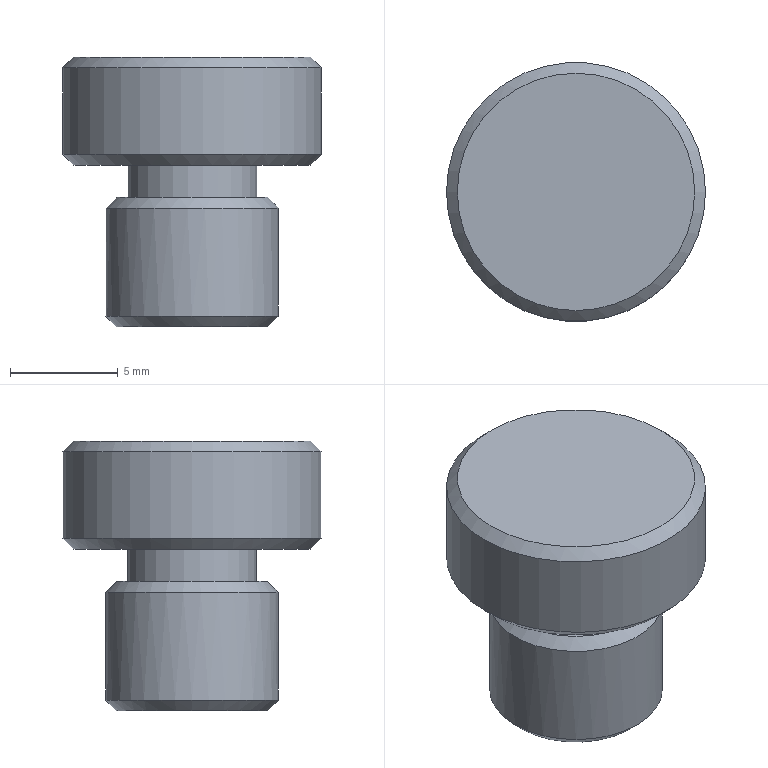Component | NX | SUPPORT_PIN_4 | 1 solid | 11 faces | box 12 x 12 x 12.5 mm | volume 894 mm3 | plane 4 | cone 4 | cylinder 3 | commonest cylinder face diameters 8 x1 6 x1 12 x1
STEP:
#1=CARTESIAN_POINT('',(0.,0.,0.));
#2=DIRECTION('',(0.,0.,1.));
#3=DIRECTION('',(1.,0.,0.));
#4=AXIS2_PLACEMENT_3D('',#1,#2,#3);
#5=CARTESIAN_POINT('',(405.601,61.,87.5));
#6=VERTEX_POINT('',#5);
#7=CARTESIAN_POINT('',(402.101,61.,87.5));
#8=DIRECTION('',(0.,0.,1.));
#9=DIRECTION('',(1.,0.,0.));
#10=AXIS2_PLACEMENT_3D('',#7,#8,#9);
#11=CIRCLE('',#10,3.5);
#12=CARTESIAN_POINT('',(402.101,61.,87.5));
#13=DIRECTION('',(0.,0.,1.));
#14=DIRECTION('',(1.,0.,0.));
#15=AXIS2_PLACEMENT_3D('',#12,#13,#14);
#16=PLANE('',#15);
#17=CARTESIAN_POINT('',(0.,0.));
#18=DIRECTION('',(1.,0.));
#19=AXIS2_PLACEMENT_2D('',#17,#18);
#20=CIRCLE('',#19,3.5);
#21=(GEOMETRIC_REPRESENTATION_CONTEXT(2)PARAMETRIC_REPRESENTATION_CONTEXT()REPRESENTATION_CONTEXT('',''));
#22=DEFINITIONAL_REPRESENTATION('',(#20),#21);
#23=PCURVE('',#16,#22);
#24=CARTESIAN_POINT('',(402.101,61.,87.));
#25=DIRECTION('',(0.,0.,-1.));
#26=DIRECTION('',(-1.,0.,0.));
#27=AXIS2_PLACEMENT_3D('',#24,#25,#26);
#28=CONICAL_SURFACE('',#27,4.,0.7854);
#29=CARTESIAN_POINT('',(9.425,-0.5));
#30=DIRECTION('',(-1.,0.));
#31=VECTOR('',#30,1.);
#32=LINE('',#29,#31);
#33=(GEOMETRIC_REPRESENTATION_CONTEXT(2)PARAMETRIC_REPRESENTATION_CONTEXT()REPRESENTATION_CONTEXT('',''));
#34=DEFINITIONAL_REPRESENTATION('',(#32),#33);
#35=PCURVE('',#28,#34);
#36=SURFACE_CURVE('',#11,(#23,#35),.PCURVE_S1.);
#37=EDGE_CURVE('',#6,#6,#36,.T.);
#38=ORIENTED_EDGE('',*,*,#37,.T.);
#39=EDGE_LOOP('',(#38));
#40=FACE_BOUND('',#39,.T.);
#41=CARTESIAN_POINT('',(405.101,61.,87.5));
#42=VERTEX_POINT('',#41);
#43=CARTESIAN_POINT('',(402.101,61.,87.5));
#44=DIRECTION('',(0.,0.,1.));
#45=DIRECTION('',(1.,0.,0.));
#46=AXIS2_PLACEMENT_3D('',#43,#44,#45);
#47=CIRCLE('',#46,3.);
#48=CARTESIAN_POINT('',(0.,0.));
#49=DIRECTION('',(1.,0.));
#50=AXIS2_PLACEMENT_2D('',#48,#49);
#51=CIRCLE('',#50,3.);
#52=(GEOMETRIC_REPRESENTATION_CONTEXT(2)PARAMETRIC_REPRESENTATION_CONTEXT()REPRESENTATION_CONTEXT('',''));
#53=DEFINITIONAL_REPRESENTATION('',(#51),#52);
#54=PCURVE('',#16,#53);
#55=CARTESIAN_POINT('',(402.101,61.,87.5));
#56=DIRECTION('',(0.,0.,1.));
#57=DIRECTION('',(1.,0.,0.));
#58=AXIS2_PLACEMENT_3D('',#55,#56,#57);
#59=CYLINDRICAL_SURFACE('',#58,3.);
#60=CARTESIAN_POINT('',(0.,0.));
#61=DIRECTION('',(1.,0.));
#62=VECTOR('',#61,1.);
#63=LINE('',#60,#62);
#64=(GEOMETRIC_REPRESENTATION_CONTEXT(2)PARAMETRIC_REPRESENTATION_CONTEXT()REPRESENTATION_CONTEXT('',''));
#65=DEFINITIONAL_REPRESENTATION('',(#63),#64);
#66=PCURVE('',#59,#65);
#67=SURFACE_CURVE('',#47,(#54,#66),.PCURVE_S1.);
#68=EDGE_CURVE('',#42,#42,#67,.T.);
#69=ORIENTED_EDGE('',*,*,#68,.F.);
#70=EDGE_LOOP('',(#69));
#71=FACE_BOUND('',#70,.T.);
#72=ADVANCED_FACE('',(#40,#71),#16,.T.);
#73=CARTESIAN_POINT('',(398.601,61.,81.5));
#74=VERTEX_POINT('',#73);
#75=CARTESIAN_POINT('',(402.101,61.,81.5));
#76=DIRECTION('',(0.,0.,-1.));
#77=DIRECTION('',(-1.,0.,0.));
#78=AXIS2_PLACEMENT_3D('',#75,#76,#77);
#79=CIRCLE('',#78,3.5);
#80=CARTESIAN_POINT('',(402.101,61.,81.5));
#81=DIRECTION('',(0.,0.,-1.));
#82=DIRECTION('',(-1.,0.,0.));
#83=AXIS2_PLACEMENT_3D('',#80,#81,#82);
#84=PLANE('',#83);
#85=CARTESIAN_POINT('',(0.,0.));
#86=DIRECTION('',(1.,0.));
#87=AXIS2_PLACEMENT_2D('',#85,#86);
#88=CIRCLE('',#87,3.5);
#89=(GEOMETRIC_REPRESENTATION_CONTEXT(2)PARAMETRIC_REPRESENTATION_CONTEXT()REPRESENTATION_CONTEXT('',''));
#90=DEFINITIONAL_REPRESENTATION('',(#88),#89);
#91=PCURVE('',#84,#90);
#92=CARTESIAN_POINT('',(402.101,61.,82.));
#93=DIRECTION('',(0.,0.,1.));
#94=DIRECTION('',(1.,0.,0.));
#95=AXIS2_PLACEMENT_3D('',#92,#93,#94);
#96=CONICAL_SURFACE('',#95,4.,0.7854);
#97=CARTESIAN_POINT('',(9.425,-0.5));
#98=DIRECTION('',(-1.,0.));
#99=VECTOR('',#98,1.);
#100=LINE('',#97,#99);
#101=(GEOMETRIC_REPRESENTATION_CONTEXT(2)PARAMETRIC_REPRESENTATION_CONTEXT()REPRESENTATION_CONTEXT('',''));
#102=DEFINITIONAL_REPRESENTATION('',(#100),#101);
#103=PCURVE('',#96,#102);
#104=SURFACE_CURVE('',#79,(#91,#103),.PCURVE_S1.);
#105=EDGE_CURVE('',#74,#74,#104,.T.);
#106=ORIENTED_EDGE('',*,*,#105,.T.);
#107=EDGE_LOOP('',(#106));
#108=FACE_BOUND('',#107,.T.);
#109=ADVANCED_FACE('',(#108),#84,.T.);
#110=CARTESIAN_POINT('',(398.101,61.,82.));
#111=VERTEX_POINT('',#110);
#112=CARTESIAN_POINT('',(406.101,61.,82.));
#113=VERTEX_POINT('',#112);
#114=CARTESIAN_POINT('',(402.101,61.,82.));
#115=DIRECTION('',(0.,0.,1.));
#116=DIRECTION('',(-1.,0.,0.));
#117=AXIS2_PLACEMENT_3D('',#114,#115,#116);
#118=CIRCLE('',#117,4.);
#119=CARTESIAN_POINT('',(402.101,61.,81.5));
#120=DIRECTION('',(0.,0.,1.));
#121=DIRECTION('',(1.,0.,0.));
#122=AXIS2_PLACEMENT_3D('',#119,#120,#121);
#123=CYLINDRICAL_SURFACE('',#122,4.);
#124=CARTESIAN_POINT('',(3.142,0.5));
#125=DIRECTION('',(1.,0.));
#126=VECTOR('',#125,1.);
#127=LINE('',#124,#126);
#128=(GEOMETRIC_REPRESENTATION_CONTEXT(2)PARAMETRIC_REPRESENTATION_CONTEXT()REPRESENTATION_CONTEXT('',''));
#129=DEFINITIONAL_REPRESENTATION('',(#127),#128);
#130=PCURVE('',#123,#129);
#131=CARTESIAN_POINT('',(3.142,0.));
#132=DIRECTION('',(1.,0.));
#133=VECTOR('',#132,1.);
#134=LINE('',#131,#133);
#135=(GEOMETRIC_REPRESENTATION_CONTEXT(2)PARAMETRIC_REPRESENTATION_CONTEXT()REPRESENTATION_CONTEXT('',''));
#136=DEFINITIONAL_REPRESENTATION('',(#134),#135);
#137=PCURVE('',#96,#136);
#138=SURFACE_CURVE('',#118,(#130,#137),.PCURVE_S1.);
#139=EDGE_CURVE('',#111,#113,#138,.T.);
#140=ORIENTED_EDGE('',*,*,#139,.T.);
#141=CARTESIAN_POINT('',(406.101,61.,87.));
#142=VERTEX_POINT('',#141);
#143=CARTESIAN_POINT('',(406.101,61.,82.));
#144=CARTESIAN_POINT('',(406.101,61.,87.));
#145=B_SPLINE_CURVE_WITH_KNOTS('',1,(#143,#144),.UNSPECIFIED.,.F.,.F.,(2,2),(0.5,5.5),.PIECEWISE_BEZIER_KNOTS.);
#146=CARTESIAN_POINT('',(6.283,0.));
#147=DIRECTION('',(0.,1.));
#148=VECTOR('',#147,1.);
#149=LINE('',#146,#148);
#150=(GEOMETRIC_REPRESENTATION_CONTEXT(2)PARAMETRIC_REPRESENTATION_CONTEXT()REPRESENTATION_CONTEXT('',''));
#151=DEFINITIONAL_REPRESENTATION('',(#149),#150);
#152=PCURVE('',#123,#151);
#153=CARTESIAN_POINT('',(0.,0.));
#154=DIRECTION('',(0.,1.));
#155=VECTOR('',#154,1.);
#156=LINE('',#153,#155);
#157=(GEOMETRIC_REPRESENTATION_CONTEXT(2)PARAMETRIC_REPRESENTATION_CONTEXT()REPRESENTATION_CONTEXT('',''));
#158=DEFINITIONAL_REPRESENTATION('',(#156),#157);
#159=PCURVE('',#123,#158);
#160=SEAM_CURVE('',#145,(#152,#159),.PCURVE_S1.);
#161=EDGE_CURVE('',#113,#142,#160,.T.);
#162=ORIENTED_EDGE('',*,*,#161,.T.);
#163=CARTESIAN_POINT('',(402.101,61.,87.));
#164=DIRECTION('',(0.,0.,-1.));
#165=DIRECTION('',(1.,0.,0.));
#166=AXIS2_PLACEMENT_3D('',#163,#164,#165);
#167=CIRCLE('',#166,4.);
#168=CARTESIAN_POINT('',(6.283,5.5));
#169=DIRECTION('',(-1.,0.));
#170=VECTOR('',#169,1.);
#171=LINE('',#168,#170);
#172=(GEOMETRIC_REPRESENTATION_CONTEXT(2)PARAMETRIC_REPRESENTATION_CONTEXT()REPRESENTATION_CONTEXT('',''));
#173=DEFINITIONAL_REPRESENTATION('',(#171),#172);
#174=PCURVE('',#123,#173);
#175=CARTESIAN_POINT('',(3.142,0.));
#176=DIRECTION('',(1.,0.));
#177=VECTOR('',#176,1.);
#178=LINE('',#175,#177);
#179=(GEOMETRIC_REPRESENTATION_CONTEXT(2)PARAMETRIC_REPRESENTATION_CONTEXT()REPRESENTATION_CONTEXT('',''));
#180=DEFINITIONAL_REPRESENTATION('',(#178),#179);
#181=PCURVE('',#28,#180);
#182=SURFACE_CURVE('',#167,(#174,#181),.PCURVE_S1.);
#183=EDGE_CURVE('',#142,#142,#182,.T.);
#184=ORIENTED_EDGE('',*,*,#183,.T.);
#185=ORIENTED_EDGE('',*,*,#161,.F.);
#186=CARTESIAN_POINT('',(402.101,61.,82.));
#187=DIRECTION('',(0.,0.,1.));
#188=DIRECTION('',(-1.,0.,0.));
#189=AXIS2_PLACEMENT_3D('',#186,#187,#188);
#190=CIRCLE('',#189,4.);
#191=CARTESIAN_POINT('',(-3.142,0.5));
#192=DIRECTION('',(1.,0.));
#193=VECTOR('',#192,1.);
#194=LINE('',#191,#193);
#195=(GEOMETRIC_REPRESENTATION_CONTEXT(2)PARAMETRIC_REPRESENTATION_CONTEXT()REPRESENTATION_CONTEXT('',''));
#196=DEFINITIONAL_REPRESENTATION('',(#194),#195);
#197=PCURVE('',#123,#196);
#198=CARTESIAN_POINT('',(3.142,0.));
#199=DIRECTION('',(1.,0.));
#200=VECTOR('',#199,1.);
#201=LINE('',#198,#200);
#202=(GEOMETRIC_REPRESENTATION_CONTEXT(2)PARAMETRIC_REPRESENTATION_CONTEXT()REPRESENTATION_CONTEXT('',''));
#203=DEFINITIONAL_REPRESENTATION('',(#201),#202);
#204=PCURVE('',#96,#203);
#205=SURFACE_CURVE('',#190,(#197,#204),.PCURVE_S1.);
#206=EDGE_CURVE('',#113,#111,#205,.T.);
#207=ORIENTED_EDGE('',*,*,#206,.T.);
#208=EDGE_LOOP('',(#140,#162,#184,#185,#207));
#209=FACE_BOUND('',#208,.T.);
#210=ADVANCED_FACE('',(#209),#123,.T.);
#211=CARTESIAN_POINT('',(405.101,61.,89.));
#212=VERTEX_POINT('',#211);
#213=CARTESIAN_POINT('',(402.101,61.,89.));
#214=DIRECTION('',(0.,0.,-1.));
#215=DIRECTION('',(1.,0.,0.));
#216=AXIS2_PLACEMENT_3D('',#213,#214,#215);
#217=CIRCLE('',#216,3.);
#218=CARTESIAN_POINT('',(6.283,1.5));
#219=DIRECTION('',(-1.,0.));
#220=VECTOR('',#219,1.);
#221=LINE('',#218,#220);
#222=(GEOMETRIC_REPRESENTATION_CONTEXT(2)PARAMETRIC_REPRESENTATION_CONTEXT()REPRESENTATION_CONTEXT('',''));
#223=DEFINITIONAL_REPRESENTATION('',(#221),#222);
#224=PCURVE('',#59,#223);
#225=CARTESIAN_POINT('',(402.101,61.,89.));
#226=DIRECTION('',(0.,0.,-1.));
#227=DIRECTION('',(-1.,0.,0.));
#228=AXIS2_PLACEMENT_3D('',#225,#226,#227);
#229=PLANE('',#228);
#230=CARTESIAN_POINT('',(0.,0.));
#231=DIRECTION('',(-1.,0.));
#232=AXIS2_PLACEMENT_2D('',#230,#231);
#233=CIRCLE('',#232,3.);
#234=(GEOMETRIC_REPRESENTATION_CONTEXT(2)PARAMETRIC_REPRESENTATION_CONTEXT()REPRESENTATION_CONTEXT('',''));
#235=DEFINITIONAL_REPRESENTATION('',(#233),#234);
#236=PCURVE('',#229,#235);
#237=SURFACE_CURVE('',#217,(#224,#236),.PCURVE_S1.);
#238=EDGE_CURVE('',#212,#212,#237,.T.);
#239=ORIENTED_EDGE('',*,*,#238,.T.);
#240=CARTESIAN_POINT('',(405.101,61.,87.5));
#241=CARTESIAN_POINT('',(405.101,61.,89.));
#242=B_SPLINE_CURVE_WITH_KNOTS('',1,(#240,#241),.UNSPECIFIED.,.F.,.F.,(2,2),(0.,1.5),.PIECEWISE_BEZIER_KNOTS.);
#243=CARTESIAN_POINT('',(0.,0.));
#244=DIRECTION('',(0.,1.));
#245=VECTOR('',#244,1.);
#246=LINE('',#243,#245);
#247=(GEOMETRIC_REPRESENTATION_CONTEXT(2)PARAMETRIC_REPRESENTATION_CONTEXT()REPRESENTATION_CONTEXT('',''));
#248=DEFINITIONAL_REPRESENTATION('',(#246),#247);
#249=PCURVE('',#59,#248);
#250=CARTESIAN_POINT('',(6.283,0.));
#251=DIRECTION('',(0.,1.));
#252=VECTOR('',#251,1.);
#253=LINE('',#250,#252);
#254=(GEOMETRIC_REPRESENTATION_CONTEXT(2)PARAMETRIC_REPRESENTATION_CONTEXT()REPRESENTATION_CONTEXT('',''));
#255=DEFINITIONAL_REPRESENTATION('',(#253),#254);
#256=PCURVE('',#59,#255);
#257=SEAM_CURVE('',#242,(#249,#256),.PCURVE_S1.);
#258=EDGE_CURVE('',#42,#212,#257,.T.);
#259=ORIENTED_EDGE('',*,*,#258,.F.);
#260=ORIENTED_EDGE('',*,*,#68,.T.);
#261=ORIENTED_EDGE('',*,*,#258,.T.);
#262=EDGE_LOOP('',(#239,#259,#260,#261));
#263=FACE_BOUND('',#262,.T.);
#264=ADVANCED_FACE('',(#263),#59,.T.);
#265=CARTESIAN_POINT('',(407.601,61.,94.));
#266=VERTEX_POINT('',#265);
#267=CARTESIAN_POINT('',(402.101,61.,94.));
#268=DIRECTION('',(0.,0.,1.));
#269=DIRECTION('',(1.,0.,0.));
#270=AXIS2_PLACEMENT_3D('',#267,#268,#269);
#271=CIRCLE('',#270,5.5);
#272=CARTESIAN_POINT('',(402.101,61.,94.));
#273=DIRECTION('',(0.,0.,1.));
#274=DIRECTION('',(1.,0.,0.));
#275=AXIS2_PLACEMENT_3D('',#272,#273,#274);
#276=PLANE('',#275);
#277=CARTESIAN_POINT('',(0.,0.));
#278=DIRECTION('',(1.,0.));
#279=AXIS2_PLACEMENT_2D('',#277,#278);
#280=CIRCLE('',#279,5.5);
#281=(GEOMETRIC_REPRESENTATION_CONTEXT(2)PARAMETRIC_REPRESENTATION_CONTEXT()REPRESENTATION_CONTEXT('',''));
#282=DEFINITIONAL_REPRESENTATION('',(#280),#281);
#283=PCURVE('',#276,#282);
#284=CARTESIAN_POINT('',(402.101,61.,93.5));
#285=DIRECTION('',(0.,0.,-1.));
#286=DIRECTION('',(-1.,0.,0.));
#287=AXIS2_PLACEMENT_3D('',#284,#285,#286);
#288=CONICAL_SURFACE('',#287,6.,0.7854);
#289=CARTESIAN_POINT('',(9.425,-0.5));
#290=DIRECTION('',(-1.,0.));
#291=VECTOR('',#290,1.);
#292=LINE('',#289,#291);
#293=(GEOMETRIC_REPRESENTATION_CONTEXT(2)PARAMETRIC_REPRESENTATION_CONTEXT()REPRESENTATION_CONTEXT('',''));
#294=DEFINITIONAL_REPRESENTATION('',(#292),#293);
#295=PCURVE('',#288,#294);
#296=SURFACE_CURVE('',#271,(#283,#295),.PCURVE_S1.);
#297=EDGE_CURVE('',#266,#266,#296,.T.);
#298=ORIENTED_EDGE('',*,*,#297,.T.);
#299=EDGE_LOOP('',(#298));
#300=FACE_BOUND('',#299,.T.);
#301=ADVANCED_FACE('',(#300),#276,.T.);
#302=CARTESIAN_POINT('',(396.601,61.,89.));
#303=VERTEX_POINT('',#302);
#304=CARTESIAN_POINT('',(402.101,61.,89.));
#305=DIRECTION('',(0.,0.,-1.));
#306=DIRECTION('',(-1.,0.,0.));
#307=AXIS2_PLACEMENT_3D('',#304,#305,#306);
#308=CIRCLE('',#307,5.5);
#309=CARTESIAN_POINT('',(0.,0.));
#310=DIRECTION('',(1.,0.));
#311=AXIS2_PLACEMENT_2D('',#309,#310);
#312=CIRCLE('',#311,5.5);
#313=(GEOMETRIC_REPRESENTATION_CONTEXT(2)PARAMETRIC_REPRESENTATION_CONTEXT()REPRESENTATION_CONTEXT('',''));
#314=DEFINITIONAL_REPRESENTATION('',(#312),#313);
#315=PCURVE('',#229,#314);
#316=CARTESIAN_POINT('',(402.101,61.,89.5));
#317=DIRECTION('',(0.,0.,1.));
#318=DIRECTION('',(1.,0.,0.));
#319=AXIS2_PLACEMENT_3D('',#316,#317,#318);
#320=CONICAL_SURFACE('',#319,6.,0.7854);
#321=CARTESIAN_POINT('',(9.425,-0.5));
#322=DIRECTION('',(-1.,0.));
#323=VECTOR('',#322,1.);
#324=LINE('',#321,#323);
#325=(GEOMETRIC_REPRESENTATION_CONTEXT(2)PARAMETRIC_REPRESENTATION_CONTEXT()REPRESENTATION_CONTEXT('',''));
#326=DEFINITIONAL_REPRESENTATION('',(#324),#325);
#327=PCURVE('',#320,#326);
#328=SURFACE_CURVE('',#308,(#315,#327),.PCURVE_S1.);
#329=EDGE_CURVE('',#303,#303,#328,.T.);
#330=ORIENTED_EDGE('',*,*,#329,.T.);
#331=EDGE_LOOP('',(#330));
#332=FACE_BOUND('',#331,.T.);
#333=ORIENTED_EDGE('',*,*,#238,.F.);
#334=EDGE_LOOP('',(#333));
#335=FACE_BOUND('',#334,.T.);
#336=ADVANCED_FACE('',(#332,#335),#229,.T.);
#337=CARTESIAN_POINT('',(396.101,61.,89.5));
#338=VERTEX_POINT('',#337);
#339=CARTESIAN_POINT('',(408.101,61.,89.5));
#340=VERTEX_POINT('',#339);
#341=CARTESIAN_POINT('',(402.101,61.,89.5));
#342=DIRECTION('',(0.,0.,1.));
#343=DIRECTION('',(-1.,0.,0.));
#344=AXIS2_PLACEMENT_3D('',#341,#342,#343);
#345=CIRCLE('',#344,6.);
#346=CARTESIAN_POINT('',(402.101,61.,89.));
#347=DIRECTION('',(0.,0.,1.));
#348=DIRECTION('',(1.,0.,0.));
#349=AXIS2_PLACEMENT_3D('',#346,#347,#348);
#350=CYLINDRICAL_SURFACE('',#349,6.);
#351=CARTESIAN_POINT('',(3.142,0.5));
#352=DIRECTION('',(1.,0.));
#353=VECTOR('',#352,1.);
#354=LINE('',#351,#353);
#355=(GEOMETRIC_REPRESENTATION_CONTEXT(2)PARAMETRIC_REPRESENTATION_CONTEXT()REPRESENTATION_CONTEXT('',''));
#356=DEFINITIONAL_REPRESENTATION('',(#354),#355);
#357=PCURVE('',#350,#356);
#358=CARTESIAN_POINT('',(3.142,0.));
#359=DIRECTION('',(1.,0.));
#360=VECTOR('',#359,1.);
#361=LINE('',#358,#360);
#362=(GEOMETRIC_REPRESENTATION_CONTEXT(2)PARAMETRIC_REPRESENTATION_CONTEXT()REPRESENTATION_CONTEXT('',''));
#363=DEFINITIONAL_REPRESENTATION('',(#361),#362);
#364=PCURVE('',#320,#363);
#365=SURFACE_CURVE('',#345,(#357,#364),.PCURVE_S1.);
#366=EDGE_CURVE('',#338,#340,#365,.T.);
#367=ORIENTED_EDGE('',*,*,#366,.T.);
#368=CARTESIAN_POINT('',(408.101,61.,93.5));
#369=VERTEX_POINT('',#368);
#370=CARTESIAN_POINT('',(408.101,61.,89.5));
#371=CARTESIAN_POINT('',(408.101,61.,93.5));
#372=B_SPLINE_CURVE_WITH_KNOTS('',1,(#370,#371),.UNSPECIFIED.,.F.,.F.,(2,2),(0.5,4.5),.PIECEWISE_BEZIER_KNOTS.);
#373=CARTESIAN_POINT('',(6.283,0.));
#374=DIRECTION('',(0.,1.));
#375=VECTOR('',#374,1.);
#376=LINE('',#373,#375);
#377=(GEOMETRIC_REPRESENTATION_CONTEXT(2)PARAMETRIC_REPRESENTATION_CONTEXT()REPRESENTATION_CONTEXT('',''));
#378=DEFINITIONAL_REPRESENTATION('',(#376),#377);
#379=PCURVE('',#350,#378);
#380=CARTESIAN_POINT('',(0.,0.));
#381=DIRECTION('',(0.,1.));
#382=VECTOR('',#381,1.);
#383=LINE('',#380,#382);
#384=(GEOMETRIC_REPRESENTATION_CONTEXT(2)PARAMETRIC_REPRESENTATION_CONTEXT()REPRESENTATION_CONTEXT('',''));
#385=DEFINITIONAL_REPRESENTATION('',(#383),#384);
#386=PCURVE('',#350,#385);
#387=SEAM_CURVE('',#372,(#379,#386),.PCURVE_S1.);
#388=EDGE_CURVE('',#340,#369,#387,.T.);
#389=ORIENTED_EDGE('',*,*,#388,.T.);
#390=CARTESIAN_POINT('',(402.101,61.,93.5));
#391=DIRECTION('',(0.,0.,-1.));
#392=DIRECTION('',(1.,0.,0.));
#393=AXIS2_PLACEMENT_3D('',#390,#391,#392);
#394=CIRCLE('',#393,6.);
#395=CARTESIAN_POINT('',(6.283,4.5));
#396=DIRECTION('',(-1.,0.));
#397=VECTOR('',#396,1.);
#398=LINE('',#395,#397);
#399=(GEOMETRIC_REPRESENTATION_CONTEXT(2)PARAMETRIC_REPRESENTATION_CONTEXT()REPRESENTATION_CONTEXT('',''));
#400=DEFINITIONAL_REPRESENTATION('',(#398),#399);
#401=PCURVE('',#350,#400);
#402=CARTESIAN_POINT('',(3.142,0.));
#403=DIRECTION('',(1.,0.));
#404=VECTOR('',#403,1.);
#405=LINE('',#402,#404);
#406=(GEOMETRIC_REPRESENTATION_CONTEXT(2)PARAMETRIC_REPRESENTATION_CONTEXT()REPRESENTATION_CONTEXT('',''));
#407=DEFINITIONAL_REPRESENTATION('',(#405),#406);
#408=PCURVE('',#288,#407);
#409=SURFACE_CURVE('',#394,(#401,#408),.PCURVE_S1.);
#410=EDGE_CURVE('',#369,#369,#409,.T.);
#411=ORIENTED_EDGE('',*,*,#410,.T.);
#412=ORIENTED_EDGE('',*,*,#388,.F.);
#413=CARTESIAN_POINT('',(402.101,61.,89.5));
#414=DIRECTION('',(0.,0.,1.));
#415=DIRECTION('',(-1.,0.,0.));
#416=AXIS2_PLACEMENT_3D('',#413,#414,#415);
#417=CIRCLE('',#416,6.);
#418=CARTESIAN_POINT('',(-3.142,0.5));
#419=DIRECTION('',(1.,0.));
#420=VECTOR('',#419,1.);
#421=LINE('',#418,#420);
#422=(GEOMETRIC_REPRESENTATION_CONTEXT(2)PARAMETRIC_REPRESENTATION_CONTEXT()REPRESENTATION_CONTEXT('',''));
#423=DEFINITIONAL_REPRESENTATION('',(#421),#422);
#424=PCURVE('',#350,#423);
#425=CARTESIAN_POINT('',(3.142,0.));
#426=DIRECTION('',(1.,0.));
#427=VECTOR('',#426,1.);
#428=LINE('',#425,#427);
#429=(GEOMETRIC_REPRESENTATION_CONTEXT(2)PARAMETRIC_REPRESENTATION_CONTEXT()REPRESENTATION_CONTEXT('',''));
#430=DEFINITIONAL_REPRESENTATION('',(#428),#429);
#431=PCURVE('',#320,#430);
#432=SURFACE_CURVE('',#417,(#424,#431),.PCURVE_S1.);
#433=EDGE_CURVE('',#340,#338,#432,.T.);
#434=ORIENTED_EDGE('',*,*,#433,.T.);
#435=EDGE_LOOP('',(#367,#389,#411,#412,#434));
#436=FACE_BOUND('',#435,.T.);
#437=ADVANCED_FACE('',(#436),#350,.T.);
#438=ORIENTED_EDGE('',*,*,#105,.F.);
#439=CARTESIAN_POINT('',(398.601,61.,81.5));
#440=CARTESIAN_POINT('',(398.101,61.,82.));
#441=B_SPLINE_CURVE_WITH_KNOTS('',1,(#439,#440),.UNSPECIFIED.,.F.,.F.,(2,2),(-0.7071,0.),.PIECEWISE_BEZIER_KNOTS.);
#442=CARTESIAN_POINT('',(9.425,0.));
#443=DIRECTION('',(0.,1.));
#444=VECTOR('',#443,1.);
#445=LINE('',#442,#444);
#446=(GEOMETRIC_REPRESENTATION_CONTEXT(2)PARAMETRIC_REPRESENTATION_CONTEXT()REPRESENTATION_CONTEXT('',''));
#447=DEFINITIONAL_REPRESENTATION('',(#445),#446);
#448=PCURVE('',#96,#447);
#449=CARTESIAN_POINT('',(3.142,0.));
#450=DIRECTION('',(0.,1.));
#451=VECTOR('',#450,1.);
#452=LINE('',#449,#451);
#453=(GEOMETRIC_REPRESENTATION_CONTEXT(2)PARAMETRIC_REPRESENTATION_CONTEXT()REPRESENTATION_CONTEXT('',''));
#454=DEFINITIONAL_REPRESENTATION('',(#452),#453);
#455=PCURVE('',#96,#454);
#456=SEAM_CURVE('',#441,(#448,#455),.PCURVE_S1.);
#457=EDGE_CURVE('',#74,#111,#456,.T.);
#458=ORIENTED_EDGE('',*,*,#457,.T.);
#459=ORIENTED_EDGE('',*,*,#206,.F.);
#460=ORIENTED_EDGE('',*,*,#139,.F.);
#461=ORIENTED_EDGE('',*,*,#457,.F.);
#462=EDGE_LOOP('',(#438,#458,#459,#460,#461));
#463=FACE_BOUND('',#462,.T.);
#464=ADVANCED_FACE('',(#463),#96,.T.);
#465=ORIENTED_EDGE('',*,*,#37,.F.);
#466=CARTESIAN_POINT('',(405.601,61.,87.5));
#467=CARTESIAN_POINT('',(406.101,61.,87.));
#468=B_SPLINE_CURVE_WITH_KNOTS('',1,(#466,#467),.UNSPECIFIED.,.F.,.F.,(2,2),(-0.7071,0.),.PIECEWISE_BEZIER_KNOTS.);
#469=CARTESIAN_POINT('',(9.425,0.));
#470=DIRECTION('',(0.,1.));
#471=VECTOR('',#470,1.);
#472=LINE('',#469,#471);
#473=(GEOMETRIC_REPRESENTATION_CONTEXT(2)PARAMETRIC_REPRESENTATION_CONTEXT()REPRESENTATION_CONTEXT('',''));
#474=DEFINITIONAL_REPRESENTATION('',(#472),#473);
#475=PCURVE('',#28,#474);
#476=CARTESIAN_POINT('',(3.142,0.));
#477=DIRECTION('',(0.,1.));
#478=VECTOR('',#477,1.);
#479=LINE('',#476,#478);
#480=(GEOMETRIC_REPRESENTATION_CONTEXT(2)PARAMETRIC_REPRESENTATION_CONTEXT()REPRESENTATION_CONTEXT('',''));
#481=DEFINITIONAL_REPRESENTATION('',(#479),#480);
#482=PCURVE('',#28,#481);
#483=SEAM_CURVE('',#468,(#475,#482),.PCURVE_S1.);
#484=EDGE_CURVE('',#6,#142,#483,.T.);
#485=ORIENTED_EDGE('',*,*,#484,.T.);
#486=ORIENTED_EDGE('',*,*,#183,.F.);
#487=ORIENTED_EDGE('',*,*,#484,.F.);
#488=EDGE_LOOP('',(#465,#485,#486,#487));
#489=FACE_BOUND('',#488,.T.);
#490=ADVANCED_FACE('',(#489),#28,.T.);
#491=ORIENTED_EDGE('',*,*,#329,.F.);
#492=CARTESIAN_POINT('',(396.601,61.,89.));
#493=CARTESIAN_POINT('',(396.101,61.,89.5));
#494=B_SPLINE_CURVE_WITH_KNOTS('',1,(#492,#493),.UNSPECIFIED.,.F.,.F.,(2,2),(-0.7071,0.),.PIECEWISE_BEZIER_KNOTS.);
#495=CARTESIAN_POINT('',(9.425,0.));
#496=DIRECTION('',(0.,1.));
#497=VECTOR('',#496,1.);
#498=LINE('',#495,#497);
#499=(GEOMETRIC_REPRESENTATION_CONTEXT(2)PARAMETRIC_REPRESENTATION_CONTEXT()REPRESENTATION_CONTEXT('',''));
#500=DEFINITIONAL_REPRESENTATION('',(#498),#499);
#501=PCURVE('',#320,#500);
#502=CARTESIAN_POINT('',(3.142,0.));
#503=DIRECTION('',(0.,1.));
#504=VECTOR('',#503,1.);
#505=LINE('',#502,#504);
#506=(GEOMETRIC_REPRESENTATION_CONTEXT(2)PARAMETRIC_REPRESENTATION_CONTEXT()REPRESENTATION_CONTEXT('',''));
#507=DEFINITIONAL_REPRESENTATION('',(#505),#506);
#508=PCURVE('',#320,#507);
#509=SEAM_CURVE('',#494,(#501,#508),.PCURVE_S1.);
#510=EDGE_CURVE('',#303,#338,#509,.T.);
#511=ORIENTED_EDGE('',*,*,#510,.T.);
#512=ORIENTED_EDGE('',*,*,#433,.F.);
#513=ORIENTED_EDGE('',*,*,#366,.F.);
#514=ORIENTED_EDGE('',*,*,#510,.F.);
#515=EDGE_LOOP('',(#491,#511,#512,#513,#514));
#516=FACE_BOUND('',#515,.T.);
#517=ADVANCED_FACE('',(#516),#320,.T.);
#518=ORIENTED_EDGE('',*,*,#297,.F.);
#519=CARTESIAN_POINT('',(407.601,61.,94.));
#520=CARTESIAN_POINT('',(408.101,61.,93.5));
#521=B_SPLINE_CURVE_WITH_KNOTS('',1,(#519,#520),.UNSPECIFIED.,.F.,.F.,(2,2),(-0.7071,0.),.PIECEWISE_BEZIER_KNOTS.);
#522=CARTESIAN_POINT('',(9.425,0.));
#523=DIRECTION('',(0.,1.));
#524=VECTOR('',#523,1.);
#525=LINE('',#522,#524);
#526=(GEOMETRIC_REPRESENTATION_CONTEXT(2)PARAMETRIC_REPRESENTATION_CONTEXT()REPRESENTATION_CONTEXT('',''));
#527=DEFINITIONAL_REPRESENTATION('',(#525),#526);
#528=PCURVE('',#288,#527);
#529=CARTESIAN_POINT('',(3.142,0.));
#530=DIRECTION('',(0.,1.));
#531=VECTOR('',#530,1.);
#532=LINE('',#529,#531);
#533=(GEOMETRIC_REPRESENTATION_CONTEXT(2)PARAMETRIC_REPRESENTATION_CONTEXT()REPRESENTATION_CONTEXT('',''));
#534=DEFINITIONAL_REPRESENTATION('',(#532),#533);
#535=PCURVE('',#288,#534);
#536=SEAM_CURVE('',#521,(#528,#535),.PCURVE_S1.);
#537=EDGE_CURVE('',#266,#369,#536,.T.);
#538=ORIENTED_EDGE('',*,*,#537,.T.);
#539=ORIENTED_EDGE('',*,*,#410,.F.);
#540=ORIENTED_EDGE('',*,*,#537,.F.);
#541=EDGE_LOOP('',(#518,#538,#539,#540));
#542=FACE_BOUND('',#541,.T.);
#543=ADVANCED_FACE('',(#542),#288,.T.);
#544=CLOSED_SHELL('',(#72,#109,#210,#264,#301,#336,#437,#464,#490,#517,#543));
#545=MANIFOLD_SOLID_BREP('',#544);
#546=(LENGTH_UNIT()NAMED_UNIT(*)SI_UNIT(.MILLI.,.METRE.));
#547=UNCERTAINTY_MEASURE_WITH_UNIT(LENGTH_MEASURE(0.00001),#546,'','');
#548=(NAMED_UNIT(*)PLANE_ANGLE_UNIT()SI_UNIT($,.RADIAN.));
#549=(NAMED_UNIT(*)SI_UNIT($,.STERADIAN.)SOLID_ANGLE_UNIT());
#550=(GEOMETRIC_REPRESENTATION_CONTEXT(3)GLOBAL_UNCERTAINTY_ASSIGNED_CONTEXT((#547))GLOBAL_UNIT_ASSIGNED_CONTEXT((#546,#548,#549))REPRESENTATION_CONTEXT('',''));
#551=ADVANCED_BREP_SHAPE_REPRESENTATION('',(#4,#545),#550);